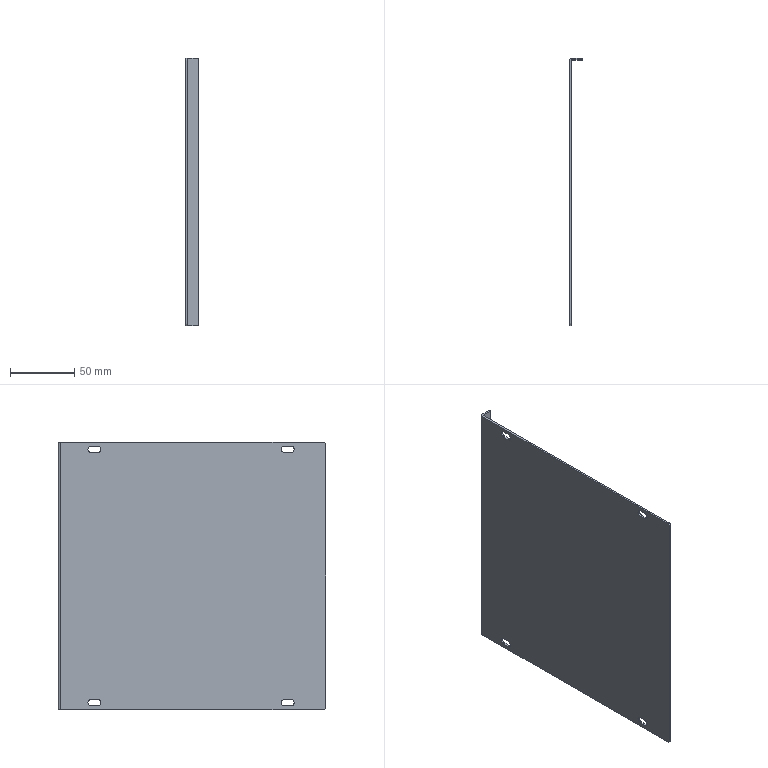Component | SolidWorks | CableEntryHoleCoverPlatePG50-104-1 | 1 solid | 40 faces | volume 66839 mm3 | plane 22 | cylinder 18 | commonest cylinder face diameters 5 x12 4 x2 5.2 x2 3.3 x1 0.3 x1 | material AISI 1045 Steel, cold drawn